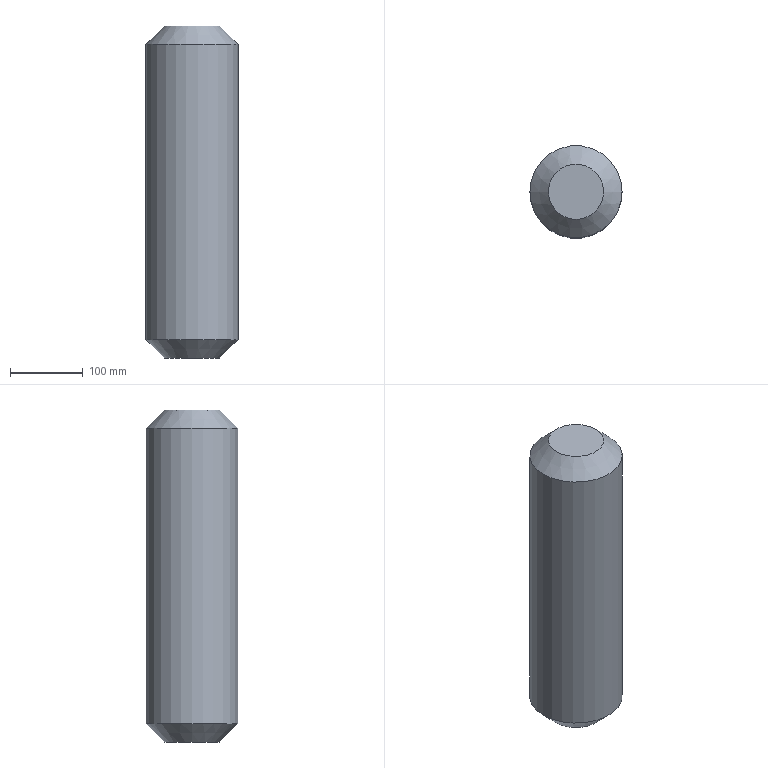Component | NX | 4_2 | 1 solid | 5 faces | volume 5568580 mm3 | plane 2 | cone 2 | cylinder 1 | commonest cylinder face diameters 127 x1